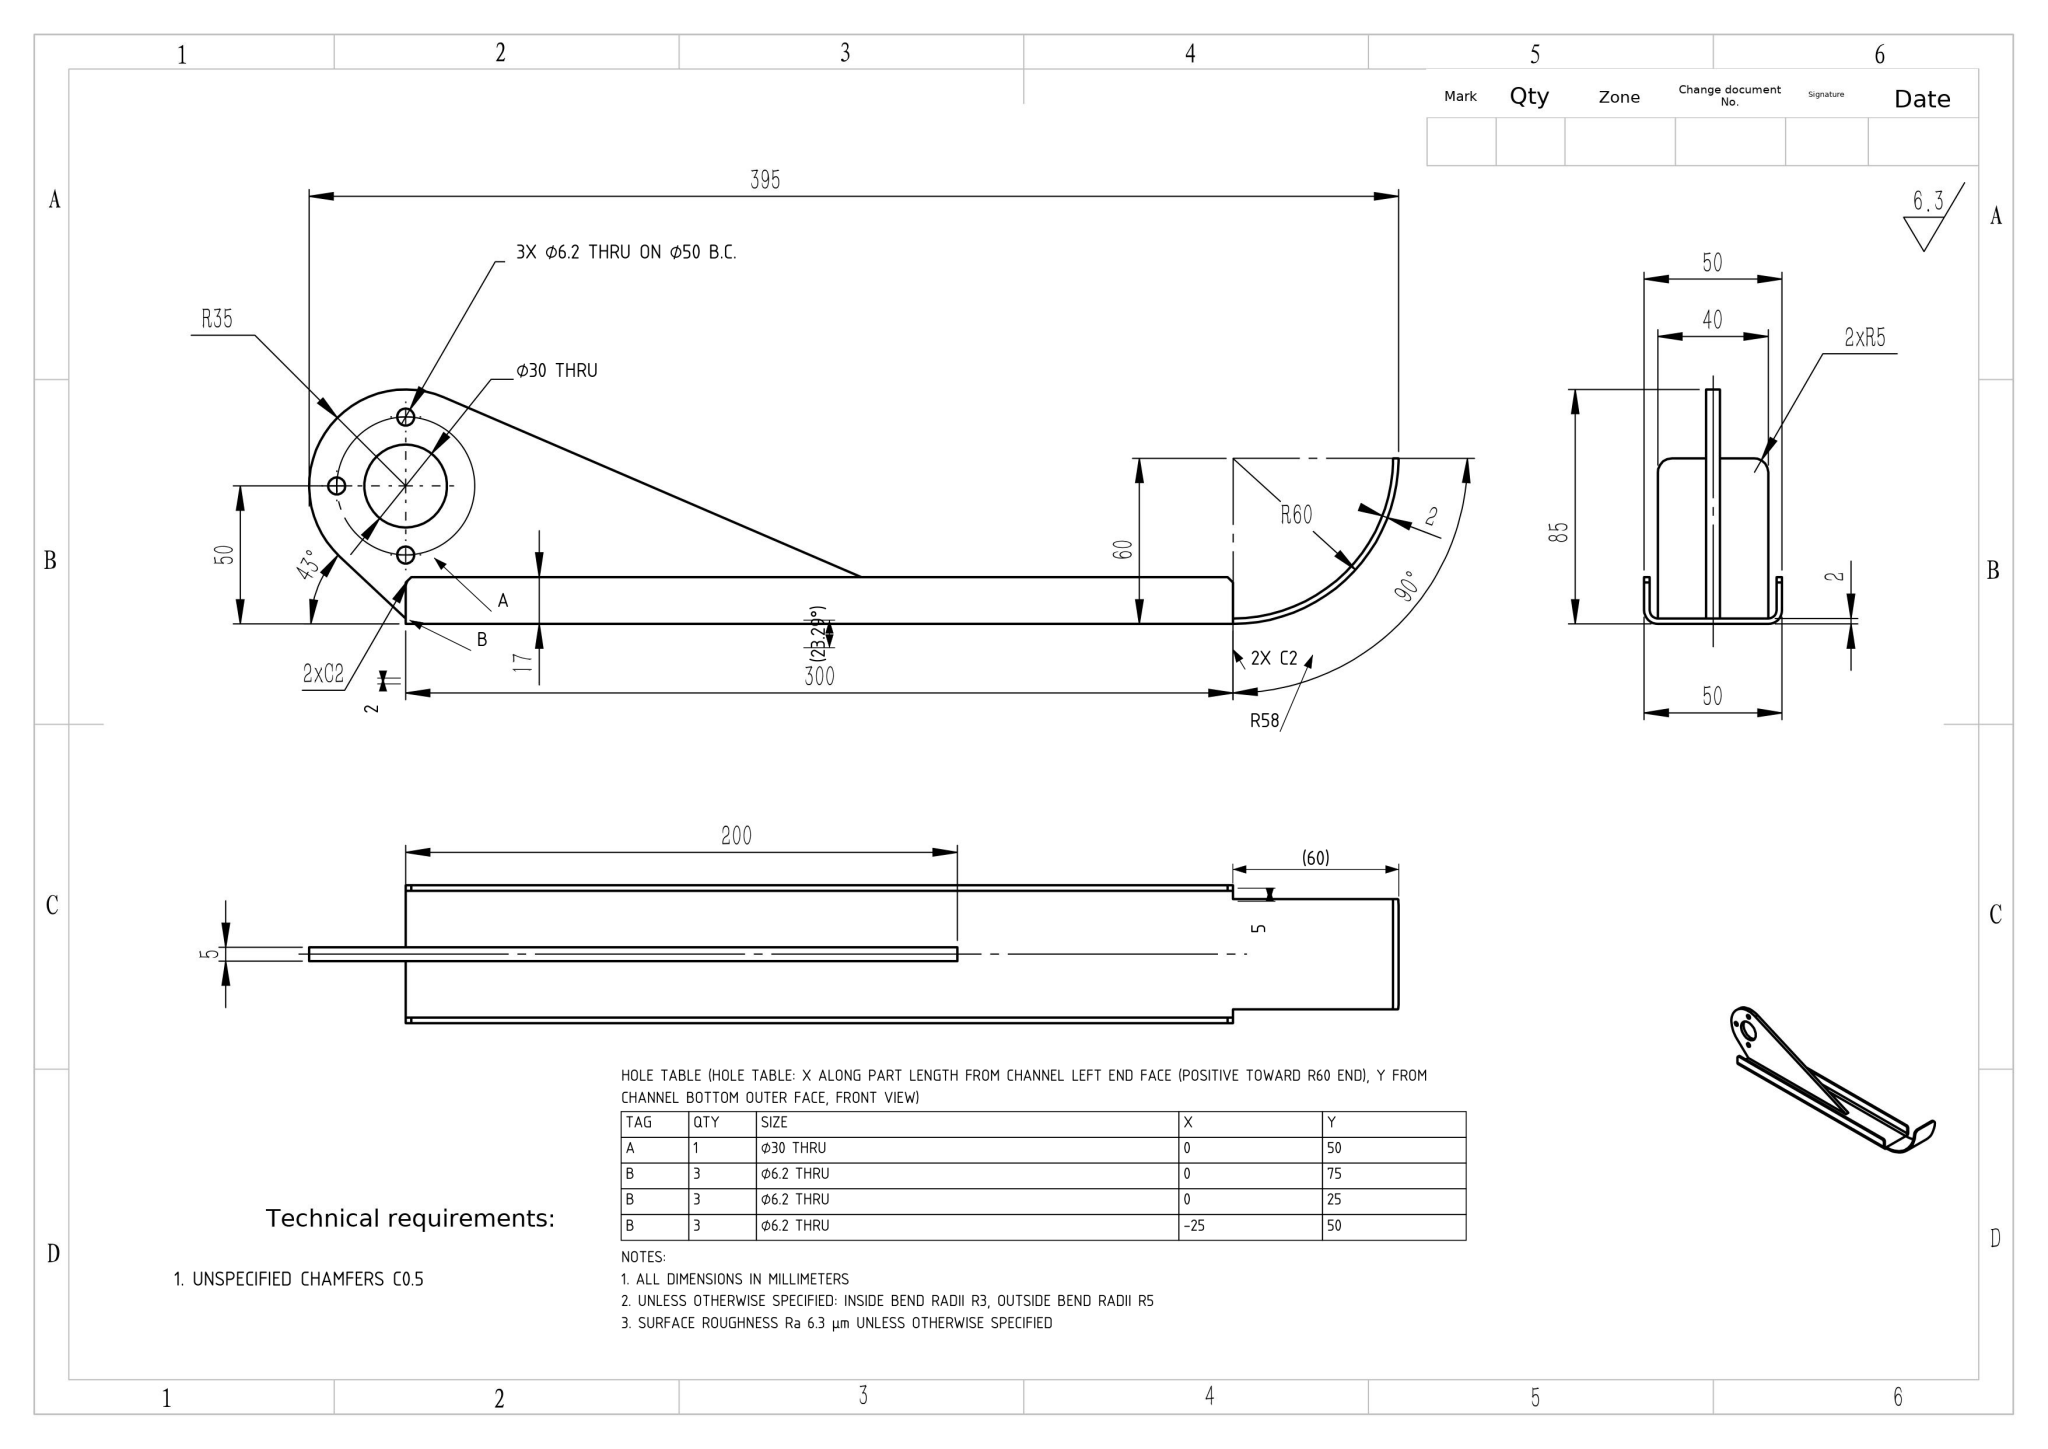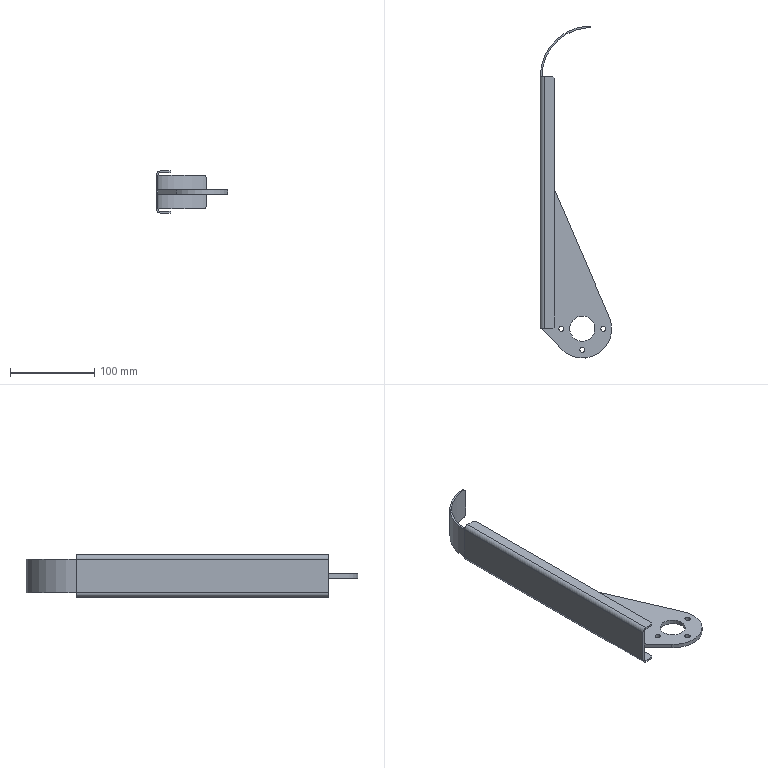Part | NX | mm | 1 solid | 45 faces | box 85 x 395 x 50 mm | volume 102496 mm3 | plane 28 | cylinder 17 | commonest cylinder face diameters 6.2 x6 10 x4 30 x2 6 x2 116 x1 120 x1 70 x1